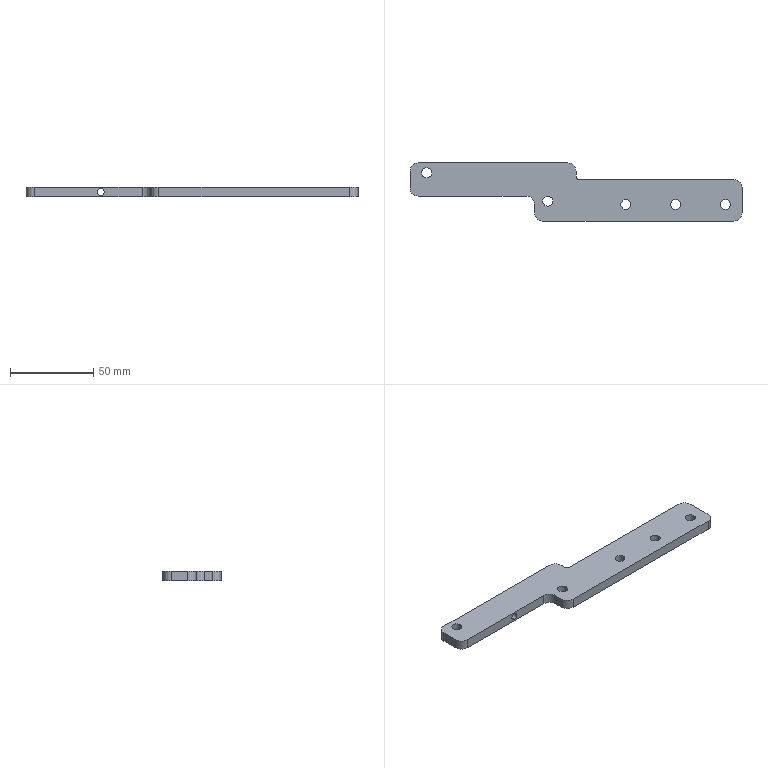Component | SolidWorks | Assembly5.1-1_MainTailstock.1-1 | 1 solid | 30 faces | box 200 x 35 x 6 mm | volume 27969 mm3 | cylinder 20 | plane 10 | commonest cylinder face diameters 6 x10 10 x7 4.2 x2 4 x1
build123d program:
from build123d import *

# Parameters (mm, degrees)
SKETCH1_R                  = 3
BOSS_EXTRUDE1_DEPTH        = 6
F_4_2_4_2_DIAMETER_HOLE1_D = 4.2


with BuildPart() as part:
    # Sketch1 → Boss-Extrude1 (new body)
    with BuildSketch(Plane.XY):
        with BuildLine():
            Line((-70, 20), (20, 20))
            ThreePointArc((20, 20), (23.536, 18.536), (25, 15))
            Line((25, 15), (25, 12))
            ThreePointArc((25, 12), (25.586, 10.586), (27, 10))
            Line((27, 10), (120, 10))
            ThreePointArc((120, 10), (123.536, 8.536), (125, 5))
            Line((125, 5), (125, -10))
            ThreePointArc((125, -10), (123.536, -13.536), (120, -15))
            Line((120, -15), (5, -15))
            ThreePointArc((5, -15), (1.464, -13.536), (0, -10))
            Line((0, -10), (0, -5))
            ThreePointArc((0, -5), (-1.464, -1.464), (-5, 0))
            Line((-5, 0), (-70, 0))
            ThreePointArc((-70, 0), (-73.536, 1.464), (-75, 5))
            Line((-75, 5), (-75, 15))
            ThreePointArc((-75, 15), (-73.536, 18.536), (-70, 20))
        make_face()
        with Locations((-65, 14)):
            Circle(SKETCH1_R, mode=Mode.SUBTRACT)
        with Locations((115, -5)):
            Circle(SKETCH1_R, mode=Mode.SUBTRACT)
        with Locations((85, -5)):
            Circle(SKETCH1_R, mode=Mode.SUBTRACT)
        with Locations((55, -5)):
            Circle(SKETCH1_R, mode=Mode.SUBTRACT)
        with Locations((8, -3)):
            Circle(SKETCH1_R, mode=Mode.SUBTRACT)
    extrude(amount=BOSS_EXTRUDE1_DEPTH)

    # 4.2 _4.2_ Diameter Hole1 (through all)
    with Locations(Plane(origin=(0, 20, 0), x_dir=(-1, 0, 0), z_dir=(0, 1, 0))):
        with Locations((30, 3)):
            Hole(F_4_2_4_2_DIAMETER_HOLE1_D / 2)


solid = part.part

# Placed as in the assembly
solid = solid.moved(Location((135, 150, -67.5), (0, 0, 0)))
STEP:
#1=COLOUR_RGB('',0.7922,0.8196,0.9333);
#2=FILL_AREA_STYLE_COLOUR('',#1);
#3=FILL_AREA_STYLE('',(#2));
#4=SURFACE_STYLE_FILL_AREA(#3);
#5=SURFACE_SIDE_STYLE('',(#4));
#6=SURFACE_STYLE_USAGE(.BOTH.,#5);
#7=PRESENTATION_STYLE_ASSIGNMENT((#6));
#8=CARTESIAN_POINT('',(4.134,5.906,-2.622));
#9=VERTEX_POINT('',#8);
#10=CARTESIAN_POINT('',(4.134,5.906,-2.457));
#11=VERTEX_POINT('',#10);
#12=CARTESIAN_POINT('',(4.134,5.906,-2.539));
#13=DIRECTION('',(-0.,1.,0.));
#14=DIRECTION('',(-1.,0.,0.));
#15=AXIS2_PLACEMENT_3D('',#12,#13,#14);
#16=CIRCLE('',#15,0.08268);
#17=EDGE_CURVE('',#9,#11,#16,.T.);
#18=ORIENTED_EDGE('',*,*,#17,.F.);
#19=CARTESIAN_POINT('',(4.134,6.693,-2.622));
#20=VERTEX_POINT('',#19);
#21=CARTESIAN_POINT('',(4.134,6.693,-2.622));
#22=DIRECTION('',(0.,1.,0.));
#23=VECTOR('',#22,39.37);
#24=LINE('',#21,#23);
#25=EDGE_CURVE('',#9,#20,#24,.T.);
#26=ORIENTED_EDGE('',*,*,#25,.T.);
#27=CARTESIAN_POINT('',(4.134,6.693,-2.457));
#28=VERTEX_POINT('',#27);
#29=CARTESIAN_POINT('',(4.134,6.693,-2.539));
#30=DIRECTION('',(0.,1.,0.));
#31=DIRECTION('',(0.,0.,1.));
#32=AXIS2_PLACEMENT_3D('',#29,#30,#31);
#33=CIRCLE('',#32,0.08268);
#34=EDGE_CURVE('',#20,#28,#33,.T.);
#35=ORIENTED_EDGE('',*,*,#34,.T.);
#36=CARTESIAN_POINT('',(4.134,6.693,-2.457));
#37=DIRECTION('',(0.,1.,0.));
#38=VECTOR('',#37,39.37);
#39=LINE('',#36,#38);
#40=EDGE_CURVE('',#11,#28,#39,.T.);
#41=ORIENTED_EDGE('',*,*,#40,.F.);
#42=EDGE_LOOP('',(#18,#26,#35,#41));
#43=FACE_OUTER_BOUND('',#42,.T.);
#44=CARTESIAN_POINT('',(4.134,6.693,-2.539));
#45=DIRECTION('',(0.,1.,0.));
#46=DIRECTION('',(0.,0.,1.));
#47=AXIS2_PLACEMENT_3D('',#44,#45,#46);
#48=CYLINDRICAL_SURFACE('',#47,0.08268);
#49=ADVANCED_FACE('',(#43),#48,.F.);
#50=CARTESIAN_POINT('',(5.512,5.787,-2.421));
#51=VERTEX_POINT('',#50);
#52=CARTESIAN_POINT('',(5.748,5.787,-2.421));
#53=VERTEX_POINT('',#52);
#54=CARTESIAN_POINT('',(5.63,5.787,-2.421));
#55=DIRECTION('',(0.,0.,1.));
#56=DIRECTION('',(1.,0.,0.));
#57=AXIS2_PLACEMENT_3D('',#54,#55,#56);
#58=CIRCLE('',#57,0.1181);
#59=EDGE_CURVE('',#51,#53,#58,.T.);
#60=ORIENTED_EDGE('',*,*,#59,.T.);
#61=CARTESIAN_POINT('',(5.748,5.787,-2.657));
#62=VERTEX_POINT('',#61);
#63=CARTESIAN_POINT('',(5.748,5.787,-2.421));
#64=DIRECTION('',(0.,0.,-1.));
#65=VECTOR('',#64,39.37);
#66=LINE('',#63,#65);
#67=EDGE_CURVE('',#53,#62,#66,.T.);
#68=ORIENTED_EDGE('',*,*,#67,.T.);
#69=CARTESIAN_POINT('',(5.512,5.787,-2.657));
#70=VERTEX_POINT('',#69);
#71=CARTESIAN_POINT('',(5.63,5.787,-2.657));
#72=DIRECTION('',(0.,0.,1.));
#73=DIRECTION('',(1.,0.,0.));
#74=AXIS2_PLACEMENT_3D('',#71,#72,#73);
#75=CIRCLE('',#74,0.1181);
#76=EDGE_CURVE('',#70,#62,#75,.T.);
#77=ORIENTED_EDGE('',*,*,#76,.F.);
#78=CARTESIAN_POINT('',(5.512,5.787,-2.421));
#79=DIRECTION('',(0.,0.,-1.));
#80=VECTOR('',#79,39.37);
#81=LINE('',#78,#80);
#82=EDGE_CURVE('',#51,#70,#81,.T.);
#83=ORIENTED_EDGE('',*,*,#82,.F.);
#84=EDGE_LOOP('',(#60,#68,#77,#83));
#85=FACE_OUTER_BOUND('',#84,.T.);
#86=CARTESIAN_POINT('',(5.63,5.787,-2.421));
#87=DIRECTION('',(0.,0.,-1.));
#88=DIRECTION('',(-1.,0.,0.));
#89=AXIS2_PLACEMENT_3D('',#86,#87,#88);
#90=CYLINDRICAL_SURFACE('',#89,0.1181);
#91=ADVANCED_FACE('',(#85),#90,.F.);
#92=CARTESIAN_POINT('',(7.362,5.709,-2.421));
#93=VERTEX_POINT('',#92);
#94=CARTESIAN_POINT('',(7.598,5.709,-2.421));
#95=VERTEX_POINT('',#94);
#96=CARTESIAN_POINT('',(7.48,5.709,-2.421));
#97=DIRECTION('',(0.,0.,1.));
#98=DIRECTION('',(1.,0.,0.));
#99=AXIS2_PLACEMENT_3D('',#96,#97,#98);
#100=CIRCLE('',#99,0.1181);
#101=EDGE_CURVE('',#93,#95,#100,.T.);
#102=ORIENTED_EDGE('',*,*,#101,.T.);
#103=CARTESIAN_POINT('',(7.598,5.709,-2.657));
#104=VERTEX_POINT('',#103);
#105=CARTESIAN_POINT('',(7.598,5.709,-2.421));
#106=DIRECTION('',(0.,0.,-1.));
#107=VECTOR('',#106,39.37);
#108=LINE('',#105,#107);
#109=EDGE_CURVE('',#95,#104,#108,.T.);
#110=ORIENTED_EDGE('',*,*,#109,.T.);
#111=CARTESIAN_POINT('',(7.362,5.709,-2.657));
#112=VERTEX_POINT('',#111);
#113=CARTESIAN_POINT('',(7.48,5.709,-2.657));
#114=DIRECTION('',(0.,0.,1.));
#115=DIRECTION('',(1.,0.,0.));
#116=AXIS2_PLACEMENT_3D('',#113,#114,#115);
#117=CIRCLE('',#116,0.1181);
#118=EDGE_CURVE('',#112,#104,#117,.T.);
#119=ORIENTED_EDGE('',*,*,#118,.F.);
#120=CARTESIAN_POINT('',(7.362,5.709,-2.421));
#121=DIRECTION('',(0.,0.,-1.));
#122=VECTOR('',#121,39.37);
#123=LINE('',#120,#122);
#124=EDGE_CURVE('',#93,#112,#123,.T.);
#125=ORIENTED_EDGE('',*,*,#124,.F.);
#126=EDGE_LOOP('',(#102,#110,#119,#125));
#127=FACE_OUTER_BOUND('',#126,.T.);
#128=CARTESIAN_POINT('',(7.48,5.709,-2.421));
#129=DIRECTION('',(0.,0.,-1.));
#130=DIRECTION('',(-1.,0.,0.));
#131=AXIS2_PLACEMENT_3D('',#128,#129,#130);
#132=CYLINDRICAL_SURFACE('',#131,0.1181);
#133=ADVANCED_FACE('',(#127),#132,.F.);
#134=CARTESIAN_POINT('',(8.543,5.709,-2.421));
#135=VERTEX_POINT('',#134);
#136=CARTESIAN_POINT('',(8.78,5.709,-2.421));
#137=VERTEX_POINT('',#136);
#138=CARTESIAN_POINT('',(8.661,5.709,-2.421));
#139=DIRECTION('',(0.,0.,1.));
#140=DIRECTION('',(1.,0.,0.));
#141=AXIS2_PLACEMENT_3D('',#138,#139,#140);
#142=CIRCLE('',#141,0.1181);
#143=EDGE_CURVE('',#135,#137,#142,.T.);
#144=ORIENTED_EDGE('',*,*,#143,.T.);
#145=CARTESIAN_POINT('',(8.78,5.709,-2.657));
#146=VERTEX_POINT('',#145);
#147=CARTESIAN_POINT('',(8.78,5.709,-2.421));
#148=DIRECTION('',(0.,0.,-1.));
#149=VECTOR('',#148,39.37);
#150=LINE('',#147,#149);
#151=EDGE_CURVE('',#137,#146,#150,.T.);
#152=ORIENTED_EDGE('',*,*,#151,.T.);
#153=CARTESIAN_POINT('',(8.543,5.709,-2.657));
#154=VERTEX_POINT('',#153);
#155=CARTESIAN_POINT('',(8.661,5.709,-2.657));
#156=DIRECTION('',(0.,0.,1.));
#157=DIRECTION('',(1.,0.,0.));
#158=AXIS2_PLACEMENT_3D('',#155,#156,#157);
#159=CIRCLE('',#158,0.1181);
#160=EDGE_CURVE('',#154,#146,#159,.T.);
#161=ORIENTED_EDGE('',*,*,#160,.F.);
#162=CARTESIAN_POINT('',(8.543,5.709,-2.421));
#163=DIRECTION('',(0.,0.,-1.));
#164=VECTOR('',#163,39.37);
#165=LINE('',#162,#164);
#166=EDGE_CURVE('',#135,#154,#165,.T.);
#167=ORIENTED_EDGE('',*,*,#166,.F.);
#168=EDGE_LOOP('',(#144,#152,#161,#167));
#169=FACE_OUTER_BOUND('',#168,.T.);
#170=CARTESIAN_POINT('',(8.661,5.709,-2.421));
#171=DIRECTION('',(0.,0.,-1.));
#172=DIRECTION('',(-1.,0.,0.));
#173=AXIS2_PLACEMENT_3D('',#170,#171,#172);
#174=CYLINDRICAL_SURFACE('',#173,0.1181);
#175=ADVANCED_FACE('',(#169),#174,.F.);
#176=CARTESIAN_POINT('',(9.724,5.709,-2.421));
#177=VERTEX_POINT('',#176);
#178=CARTESIAN_POINT('',(9.961,5.709,-2.421));
#179=VERTEX_POINT('',#178);
#180=CARTESIAN_POINT('',(9.843,5.709,-2.421));
#181=DIRECTION('',(0.,0.,1.));
#182=DIRECTION('',(1.,0.,0.));
#183=AXIS2_PLACEMENT_3D('',#180,#181,#182);
#184=CIRCLE('',#183,0.1181);
#185=EDGE_CURVE('',#177,#179,#184,.T.);
#186=ORIENTED_EDGE('',*,*,#185,.T.);
#187=CARTESIAN_POINT('',(9.961,5.709,-2.657));
#188=VERTEX_POINT('',#187);
#189=CARTESIAN_POINT('',(9.961,5.709,-2.421));
#190=DIRECTION('',(0.,0.,-1.));
#191=VECTOR('',#190,39.37);
#192=LINE('',#189,#191);
#193=EDGE_CURVE('',#179,#188,#192,.T.);
#194=ORIENTED_EDGE('',*,*,#193,.T.);
#195=CARTESIAN_POINT('',(9.724,5.709,-2.657));
#196=VERTEX_POINT('',#195);
#197=CARTESIAN_POINT('',(9.843,5.709,-2.657));
#198=DIRECTION('',(0.,0.,1.));
#199=DIRECTION('',(1.,0.,0.));
#200=AXIS2_PLACEMENT_3D('',#197,#198,#199);
#201=CIRCLE('',#200,0.1181);
#202=EDGE_CURVE('',#196,#188,#201,.T.);
#203=ORIENTED_EDGE('',*,*,#202,.F.);
#204=CARTESIAN_POINT('',(9.724,5.709,-2.421));
#205=DIRECTION('',(0.,0.,-1.));
#206=VECTOR('',#205,39.37);
#207=LINE('',#204,#206);
#208=EDGE_CURVE('',#177,#196,#207,.T.);
#209=ORIENTED_EDGE('',*,*,#208,.F.);
#210=EDGE_LOOP('',(#186,#194,#203,#209));
#211=FACE_OUTER_BOUND('',#210,.T.);
#212=CARTESIAN_POINT('',(9.843,5.709,-2.421));
#213=DIRECTION('',(0.,0.,-1.));
#214=DIRECTION('',(-1.,0.,0.));
#215=AXIS2_PLACEMENT_3D('',#212,#213,#214);
#216=CYLINDRICAL_SURFACE('',#215,0.1181);
#217=ADVANCED_FACE('',(#211),#216,.F.);
#218=CARTESIAN_POINT('',(2.638,6.457,-2.421));
#219=VERTEX_POINT('',#218);
#220=CARTESIAN_POINT('',(2.874,6.457,-2.421));
#221=VERTEX_POINT('',#220);
#222=CARTESIAN_POINT('',(2.756,6.457,-2.421));
#223=DIRECTION('',(0.,0.,1.));
#224=DIRECTION('',(1.,0.,0.));
#225=AXIS2_PLACEMENT_3D('',#222,#223,#224);
#226=CIRCLE('',#225,0.1181);
#227=EDGE_CURVE('',#219,#221,#226,.T.);
#228=ORIENTED_EDGE('',*,*,#227,.T.);
#229=CARTESIAN_POINT('',(2.874,6.457,-2.657));
#230=VERTEX_POINT('',#229);
#231=CARTESIAN_POINT('',(2.874,6.457,-2.421));
#232=DIRECTION('',(0.,0.,-1.));
#233=VECTOR('',#232,39.37);
#234=LINE('',#231,#233);
#235=EDGE_CURVE('',#221,#230,#234,.T.);
#236=ORIENTED_EDGE('',*,*,#235,.T.);
#237=CARTESIAN_POINT('',(2.638,6.457,-2.657));
#238=VERTEX_POINT('',#237);
#239=CARTESIAN_POINT('',(2.756,6.457,-2.657));
#240=DIRECTION('',(0.,0.,1.));
#241=DIRECTION('',(1.,0.,0.));
#242=AXIS2_PLACEMENT_3D('',#239,#240,#241);
#243=CIRCLE('',#242,0.1181);
#244=EDGE_CURVE('',#238,#230,#243,.T.);
#245=ORIENTED_EDGE('',*,*,#244,.F.);
#246=CARTESIAN_POINT('',(2.638,6.457,-2.421));
#247=DIRECTION('',(0.,0.,-1.));
#248=VECTOR('',#247,39.37);
#249=LINE('',#246,#248);
#250=EDGE_CURVE('',#219,#238,#249,.T.);
#251=ORIENTED_EDGE('',*,*,#250,.F.);
#252=EDGE_LOOP('',(#228,#236,#245,#251));
#253=FACE_OUTER_BOUND('',#252,.T.);
#254=CARTESIAN_POINT('',(2.756,6.457,-2.421));
#255=DIRECTION('',(0.,0.,-1.));
#256=DIRECTION('',(-1.,0.,0.));
#257=AXIS2_PLACEMENT_3D('',#254,#255,#256);
#258=CYLINDRICAL_SURFACE('',#257,0.1181);
#259=ADVANCED_FACE('',(#253),#258,.F.);
#260=ORIENTED_EDGE('',*,*,#101,.F.);
#261=CARTESIAN_POINT('',(7.48,5.709,-2.421));
#262=DIRECTION('',(0.,0.,1.));
#263=DIRECTION('',(1.,0.,0.));
#264=AXIS2_PLACEMENT_3D('',#261,#262,#263);
#265=CIRCLE('',#264,0.1181);
#266=EDGE_CURVE('',#95,#93,#265,.T.);
#267=ORIENTED_EDGE('',*,*,#266,.F.);
#268=EDGE_LOOP('',(#260,#267));
#269=FACE_BOUND('',#268,.T.);
#270=ORIENTED_EDGE('',*,*,#185,.F.);
#271=CARTESIAN_POINT('',(9.843,5.709,-2.421));
#272=DIRECTION('',(0.,0.,1.));
#273=DIRECTION('',(1.,0.,0.));
#274=AXIS2_PLACEMENT_3D('',#271,#272,#273);
#275=CIRCLE('',#274,0.1181);
#276=EDGE_CURVE('',#179,#177,#275,.T.);
#277=ORIENTED_EDGE('',*,*,#276,.F.);
#278=EDGE_LOOP('',(#270,#277));
#279=FACE_BOUND('',#278,.T.);
#280=CARTESIAN_POINT('',(10.039,5.315,-2.421));
#281=VERTEX_POINT('',#280);
#282=CARTESIAN_POINT('',(10.236,5.512,-2.421));
#283=VERTEX_POINT('',#282);
#284=CARTESIAN_POINT('',(10.039,5.512,-2.421));
#285=DIRECTION('',(0.,0.,1.));
#286=DIRECTION('',(1.,0.,0.));
#287=AXIS2_PLACEMENT_3D('',#284,#285,#286);
#288=CIRCLE('',#287,0.1969);
#289=EDGE_CURVE('',#281,#283,#288,.T.);
#290=ORIENTED_EDGE('',*,*,#289,.T.);
#291=CARTESIAN_POINT('',(10.236,6.102,-2.421));
#292=VERTEX_POINT('',#291);
#293=CARTESIAN_POINT('',(10.236,6.102,-2.421));
#294=DIRECTION('',(0.,1.,0.));
#295=VECTOR('',#294,39.37);
#296=LINE('',#293,#295);
#297=EDGE_CURVE('',#283,#292,#296,.T.);
#298=ORIENTED_EDGE('',*,*,#297,.T.);
#299=CARTESIAN_POINT('',(10.039,6.299,-2.421));
#300=VERTEX_POINT('',#299);
#301=CARTESIAN_POINT('',(10.039,6.102,-2.421));
#302=DIRECTION('',(0.,0.,1.));
#303=DIRECTION('',(1.,0.,0.));
#304=AXIS2_PLACEMENT_3D('',#301,#302,#303);
#305=CIRCLE('',#304,0.1969);
#306=EDGE_CURVE('',#292,#300,#305,.T.);
#307=ORIENTED_EDGE('',*,*,#306,.T.);
#308=CARTESIAN_POINT('',(6.378,6.299,-2.421));
#309=VERTEX_POINT('',#308);
#310=CARTESIAN_POINT('',(6.378,6.299,-2.421));
#311=DIRECTION('',(-1.,-0.,0.));
#312=VECTOR('',#311,39.37);
#313=LINE('',#310,#312);
#314=EDGE_CURVE('',#300,#309,#313,.T.);
#315=ORIENTED_EDGE('',*,*,#314,.T.);
#316=CARTESIAN_POINT('',(6.299,6.378,-2.421));
#317=VERTEX_POINT('',#316);
#318=CARTESIAN_POINT('',(6.378,6.378,-2.421));
#319=DIRECTION('',(0.,0.,-1.));
#320=DIRECTION('',(-1.,0.,0.));
#321=AXIS2_PLACEMENT_3D('',#318,#319,#320);
#322=CIRCLE('',#321,0.07874);
#323=EDGE_CURVE('',#309,#317,#322,.T.);
#324=ORIENTED_EDGE('',*,*,#323,.T.);
#325=CARTESIAN_POINT('',(6.299,6.496,-2.421));
#326=VERTEX_POINT('',#325);
#327=CARTESIAN_POINT('',(6.299,6.496,-2.421));
#328=DIRECTION('',(0.,1.,0.));
#329=VECTOR('',#328,39.37);
#330=LINE('',#327,#329);
#331=EDGE_CURVE('',#317,#326,#330,.T.);
#332=ORIENTED_EDGE('',*,*,#331,.T.);
#333=CARTESIAN_POINT('',(6.102,6.693,-2.421));
#334=VERTEX_POINT('',#333);
#335=CARTESIAN_POINT('',(6.102,6.496,-2.421));
#336=DIRECTION('',(0.,0.,1.));
#337=DIRECTION('',(1.,0.,0.));
#338=AXIS2_PLACEMENT_3D('',#335,#336,#337);
#339=CIRCLE('',#338,0.1969);
#340=EDGE_CURVE('',#326,#334,#339,.T.);
#341=ORIENTED_EDGE('',*,*,#340,.T.);
#342=CARTESIAN_POINT('',(2.559,6.693,-2.421));
#343=VERTEX_POINT('',#342);
#344=CARTESIAN_POINT('',(2.559,6.693,-2.421));
#345=DIRECTION('',(-1.,0.,0.));
#346=VECTOR('',#345,39.37);
#347=LINE('',#344,#346);
#348=EDGE_CURVE('',#334,#343,#347,.T.);
#349=ORIENTED_EDGE('',*,*,#348,.T.);
#350=CARTESIAN_POINT('',(2.362,6.496,-2.421));
#351=VERTEX_POINT('',#350);
#352=CARTESIAN_POINT('',(2.559,6.496,-2.421));
#353=DIRECTION('',(0.,0.,1.));
#354=DIRECTION('',(1.,0.,0.));
#355=AXIS2_PLACEMENT_3D('',#352,#353,#354);
#356=CIRCLE('',#355,0.1969);
#357=EDGE_CURVE('',#343,#351,#356,.T.);
#358=ORIENTED_EDGE('',*,*,#357,.T.);
#359=CARTESIAN_POINT('',(2.362,6.102,-2.421));
#360=VERTEX_POINT('',#359);
#361=CARTESIAN_POINT('',(2.362,6.102,-2.421));
#362=DIRECTION('',(0.,-1.,0.));
#363=VECTOR('',#362,39.37);
#364=LINE('',#361,#363);
#365=EDGE_CURVE('',#351,#360,#364,.T.);
#366=ORIENTED_EDGE('',*,*,#365,.T.);
#367=CARTESIAN_POINT('',(2.559,5.906,-2.421));
#368=VERTEX_POINT('',#367);
#369=CARTESIAN_POINT('',(2.559,6.102,-2.421));
#370=DIRECTION('',(0.,0.,1.));
#371=DIRECTION('',(-1.,0.,0.));
#372=AXIS2_PLACEMENT_3D('',#369,#370,#371);
#373=CIRCLE('',#372,0.1969);
#374=EDGE_CURVE('',#360,#368,#373,.T.);
#375=ORIENTED_EDGE('',*,*,#374,.T.);
#376=CARTESIAN_POINT('',(5.118,5.906,-2.421));
#377=VERTEX_POINT('',#376);
#378=CARTESIAN_POINT('',(5.118,5.906,-2.421));
#379=DIRECTION('',(1.,0.,0.));
#380=VECTOR('',#379,39.37);
#381=LINE('',#378,#380);
#382=EDGE_CURVE('',#368,#377,#381,.T.);
#383=ORIENTED_EDGE('',*,*,#382,.T.);
#384=CARTESIAN_POINT('',(5.315,5.709,-2.421));
#385=VERTEX_POINT('',#384);
#386=CARTESIAN_POINT('',(5.118,5.709,-2.421));
#387=DIRECTION('',(0.,0.,-1.));
#388=DIRECTION('',(1.,0.,0.));
#389=AXIS2_PLACEMENT_3D('',#386,#387,#388);
#390=CIRCLE('',#389,0.1969);
#391=EDGE_CURVE('',#377,#385,#390,.T.);
#392=ORIENTED_EDGE('',*,*,#391,.T.);
#393=CARTESIAN_POINT('',(5.315,5.512,-2.421));
#394=VERTEX_POINT('',#393);
#395=CARTESIAN_POINT('',(5.315,5.512,-2.421));
#396=DIRECTION('',(0.,-1.,0.));
#397=VECTOR('',#396,39.37);
#398=LINE('',#395,#397);
#399=EDGE_CURVE('',#385,#394,#398,.T.);
#400=ORIENTED_EDGE('',*,*,#399,.T.);
#401=CARTESIAN_POINT('',(5.512,5.315,-2.421));
#402=VERTEX_POINT('',#401);
#403=CARTESIAN_POINT('',(5.512,5.512,-2.421));
#404=DIRECTION('',(0.,0.,1.));
#405=DIRECTION('',(-1.,0.,0.));
#406=AXIS2_PLACEMENT_3D('',#403,#404,#405);
#407=CIRCLE('',#406,0.1969);
#408=EDGE_CURVE('',#394,#402,#407,.T.);
#409=ORIENTED_EDGE('',*,*,#408,.T.);
#410=CARTESIAN_POINT('',(10.039,5.315,-2.421));
#411=DIRECTION('',(1.,0.,0.));
#412=VECTOR('',#411,39.37);
#413=LINE('',#410,#412);
#414=EDGE_CURVE('',#402,#281,#413,.T.);
#415=ORIENTED_EDGE('',*,*,#414,.T.);
#416=EDGE_LOOP('',(#290,#298,#307,#315,#324,#332,#341,#349,#358,#366,#375,#383,#392,#400,#409,#415));
#417=FACE_OUTER_BOUND('',#416,.T.);
#418=ORIENTED_EDGE('',*,*,#227,.F.);
#419=CARTESIAN_POINT('',(2.756,6.457,-2.421));
#420=DIRECTION('',(0.,0.,1.));
#421=DIRECTION('',(1.,0.,0.));
#422=AXIS2_PLACEMENT_3D('',#419,#420,#421);
#423=CIRCLE('',#422,0.1181);
#424=EDGE_CURVE('',#221,#219,#423,.T.);
#425=ORIENTED_EDGE('',*,*,#424,.F.);
#426=EDGE_LOOP('',(#418,#425));
#427=FACE_BOUND('',#426,.T.);
#428=ORIENTED_EDGE('',*,*,#143,.F.);
#429=CARTESIAN_POINT('',(8.661,5.709,-2.421));
#430=DIRECTION('',(0.,0.,1.));
#431=DIRECTION('',(1.,0.,0.));
#432=AXIS2_PLACEMENT_3D('',#429,#430,#431);
#433=CIRCLE('',#432,0.1181);
#434=EDGE_CURVE('',#137,#135,#433,.T.);
#435=ORIENTED_EDGE('',*,*,#434,.F.);
#436=EDGE_LOOP('',(#428,#435));
#437=FACE_BOUND('',#436,.T.);
#438=ORIENTED_EDGE('',*,*,#59,.F.);
#439=CARTESIAN_POINT('',(5.63,5.787,-2.421));
#440=DIRECTION('',(0.,0.,1.));
#441=DIRECTION('',(1.,0.,0.));
#442=AXIS2_PLACEMENT_3D('',#439,#440,#441);
#443=CIRCLE('',#442,0.1181);
#444=EDGE_CURVE('',#53,#51,#443,.T.);
#445=ORIENTED_EDGE('',*,*,#444,.F.);
#446=EDGE_LOOP('',(#438,#445));
#447=FACE_BOUND('',#446,.T.);
#448=CARTESIAN_POINT('',(10.039,5.512,-2.421));
#449=DIRECTION('',(0.,0.,1.));
#450=DIRECTION('',(1.,0.,0.));
#451=AXIS2_PLACEMENT_3D('',#448,#449,#450);
#452=PLANE('',#451);
#453=ADVANCED_FACE('',(#269,#279,#417,#427,#437,#447),#452,.T.);
#454=ORIENTED_EDGE('',*,*,#118,.T.);
#455=CARTESIAN_POINT('',(7.48,5.709,-2.657));
#456=DIRECTION('',(0.,0.,1.));
#457=DIRECTION('',(1.,0.,0.));
#458=AXIS2_PLACEMENT_3D('',#455,#456,#457);
#459=CIRCLE('',#458,0.1181);
#460=EDGE_CURVE('',#104,#112,#459,.T.);
#461=ORIENTED_EDGE('',*,*,#460,.T.);
#462=EDGE_LOOP('',(#454,#461));
#463=FACE_BOUND('',#462,.T.);
#464=ORIENTED_EDGE('',*,*,#202,.T.);
#465=CARTESIAN_POINT('',(9.843,5.709,-2.657));
#466=DIRECTION('',(0.,0.,1.));
#467=DIRECTION('',(1.,0.,0.));
#468=AXIS2_PLACEMENT_3D('',#465,#466,#467);
#469=CIRCLE('',#468,0.1181);
#470=EDGE_CURVE('',#188,#196,#469,.T.);
#471=ORIENTED_EDGE('',*,*,#470,.T.);
#472=EDGE_LOOP('',(#464,#471));
#473=FACE_BOUND('',#472,.T.);
#474=CARTESIAN_POINT('',(10.039,5.315,-2.657));
#475=VERTEX_POINT('',#474);
#476=CARTESIAN_POINT('',(10.236,5.512,-2.657));
#477=VERTEX_POINT('',#476);
#478=CARTESIAN_POINT('',(10.039,5.512,-2.657));
#479=DIRECTION('',(0.,0.,1.));
#480=DIRECTION('',(1.,0.,0.));
#481=AXIS2_PLACEMENT_3D('',#478,#479,#480);
#482=CIRCLE('',#481,0.1969);
#483=EDGE_CURVE('',#475,#477,#482,.T.);
#484=ORIENTED_EDGE('',*,*,#483,.F.);
#485=CARTESIAN_POINT('',(5.512,5.315,-2.657));
#486=VERTEX_POINT('',#485);
#487=CARTESIAN_POINT('',(10.039,5.315,-2.657));
#488=DIRECTION('',(1.,0.,0.));
#489=VECTOR('',#488,39.37);
#490=LINE('',#487,#489);
#491=EDGE_CURVE('',#486,#475,#490,.T.);
#492=ORIENTED_EDGE('',*,*,#491,.F.);
#493=CARTESIAN_POINT('',(5.315,5.512,-2.657));
#494=VERTEX_POINT('',#493);
#495=CARTESIAN_POINT('',(5.512,5.512,-2.657));
#496=DIRECTION('',(0.,0.,1.));
#497=DIRECTION('',(-1.,0.,0.));
#498=AXIS2_PLACEMENT_3D('',#495,#496,#497);
#499=CIRCLE('',#498,0.1969);
#500=EDGE_CURVE('',#494,#486,#499,.T.);
#501=ORIENTED_EDGE('',*,*,#500,.F.);
#502=CARTESIAN_POINT('',(5.315,5.709,-2.657));
#503=VERTEX_POINT('',#502);
#504=CARTESIAN_POINT('',(5.315,5.512,-2.657));
#505=DIRECTION('',(0.,-1.,0.));
#506=VECTOR('',#505,39.37);
#507=LINE('',#504,#506);
#508=EDGE_CURVE('',#503,#494,#507,.T.);
#509=ORIENTED_EDGE('',*,*,#508,.F.);
#510=CARTESIAN_POINT('',(5.118,5.906,-2.657));
#511=VERTEX_POINT('',#510);
#512=CARTESIAN_POINT('',(5.118,5.709,-2.657));
#513=DIRECTION('',(0.,0.,-1.));
#514=DIRECTION('',(1.,0.,0.));
#515=AXIS2_PLACEMENT_3D('',#512,#513,#514);
#516=CIRCLE('',#515,0.1969);
#517=EDGE_CURVE('',#511,#503,#516,.T.);
#518=ORIENTED_EDGE('',*,*,#517,.F.);
#519=CARTESIAN_POINT('',(2.559,5.906,-2.657));
#520=VERTEX_POINT('',#519);
#521=CARTESIAN_POINT('',(5.118,5.906,-2.657));
#522=DIRECTION('',(1.,0.,0.));
#523=VECTOR('',#522,39.37);
#524=LINE('',#521,#523);
#525=EDGE_CURVE('',#520,#511,#524,.T.);
#526=ORIENTED_EDGE('',*,*,#525,.F.);
#527=CARTESIAN_POINT('',(2.362,6.102,-2.657));
#528=VERTEX_POINT('',#527);
#529=CARTESIAN_POINT('',(2.559,6.102,-2.657));
#530=DIRECTION('',(0.,0.,1.));
#531=DIRECTION('',(-1.,0.,0.));
#532=AXIS2_PLACEMENT_3D('',#529,#530,#531);
#533=CIRCLE('',#532,0.1969);
#534=EDGE_CURVE('',#528,#520,#533,.T.);
#535=ORIENTED_EDGE('',*,*,#534,.F.);
#536=CARTESIAN_POINT('',(2.362,6.496,-2.657));
#537=VERTEX_POINT('',#536);
#538=CARTESIAN_POINT('',(2.362,6.102,-2.657));
#539=DIRECTION('',(0.,-1.,0.));
#540=VECTOR('',#539,39.37);
#541=LINE('',#538,#540);
#542=EDGE_CURVE('',#537,#528,#541,.T.);
#543=ORIENTED_EDGE('',*,*,#542,.F.);
#544=CARTESIAN_POINT('',(2.559,6.693,-2.657));
#545=VERTEX_POINT('',#544);
#546=CARTESIAN_POINT('',(2.559,6.496,-2.657));
#547=DIRECTION('',(0.,0.,1.));
#548=DIRECTION('',(1.,0.,0.));
#549=AXIS2_PLACEMENT_3D('',#546,#547,#548);
#550=CIRCLE('',#549,0.1969);
#551=EDGE_CURVE('',#545,#537,#550,.T.);
#552=ORIENTED_EDGE('',*,*,#551,.F.);
#553=CARTESIAN_POINT('',(6.102,6.693,-2.657));
#554=VERTEX_POINT('',#553);
#555=CARTESIAN_POINT('',(2.559,6.693,-2.657));
#556=DIRECTION('',(-1.,0.,0.));
#557=VECTOR('',#556,39.37);
#558=LINE('',#555,#557);
#559=EDGE_CURVE('',#554,#545,#558,.T.);
#560=ORIENTED_EDGE('',*,*,#559,.F.);
#561=CARTESIAN_POINT('',(6.299,6.496,-2.657));
#562=VERTEX_POINT('',#561);
#563=CARTESIAN_POINT('',(6.102,6.496,-2.657));
#564=DIRECTION('',(0.,0.,1.));
#565=DIRECTION('',(1.,0.,0.));
#566=AXIS2_PLACEMENT_3D('',#563,#564,#565);
#567=CIRCLE('',#566,0.1969);
#568=EDGE_CURVE('',#562,#554,#567,.T.);
#569=ORIENTED_EDGE('',*,*,#568,.F.);
#570=CARTESIAN_POINT('',(6.299,6.378,-2.657));
#571=VERTEX_POINT('',#570);
#572=CARTESIAN_POINT('',(6.299,6.496,-2.657));
#573=DIRECTION('',(0.,1.,0.));
#574=VECTOR('',#573,39.37);
#575=LINE('',#572,#574);
#576=EDGE_CURVE('',#571,#562,#575,.T.);
#577=ORIENTED_EDGE('',*,*,#576,.F.);
#578=CARTESIAN_POINT('',(6.378,6.299,-2.657));
#579=VERTEX_POINT('',#578);
#580=CARTESIAN_POINT('',(6.378,6.378,-2.657));
#581=DIRECTION('',(0.,0.,-1.));
#582=DIRECTION('',(-1.,0.,0.));
#583=AXIS2_PLACEMENT_3D('',#580,#581,#582);
#584=CIRCLE('',#583,0.07874);
#585=EDGE_CURVE('',#579,#571,#584,.T.);
#586=ORIENTED_EDGE('',*,*,#585,.F.);
#587=CARTESIAN_POINT('',(10.039,6.299,-2.657));
#588=VERTEX_POINT('',#587);
#589=CARTESIAN_POINT('',(6.378,6.299,-2.657));
#590=DIRECTION('',(-1.,-0.,0.));
#591=VECTOR('',#590,39.37);
#592=LINE('',#589,#591);
#593=EDGE_CURVE('',#588,#579,#592,.T.);
#594=ORIENTED_EDGE('',*,*,#593,.F.);
#595=CARTESIAN_POINT('',(10.236,6.102,-2.657));
#596=VERTEX_POINT('',#595);
#597=CARTESIAN_POINT('',(10.039,6.102,-2.657));
#598=DIRECTION('',(0.,0.,1.));
#599=DIRECTION('',(1.,0.,0.));
#600=AXIS2_PLACEMENT_3D('',#597,#598,#599);
#601=CIRCLE('',#600,0.1969);
#602=EDGE_CURVE('',#596,#588,#601,.T.);
#603=ORIENTED_EDGE('',*,*,#602,.F.);
#604=CARTESIAN_POINT('',(10.236,6.102,-2.657));
#605=DIRECTION('',(0.,1.,0.));
#606=VECTOR('',#605,39.37);
#607=LINE('',#604,#606);
#608=EDGE_CURVE('',#477,#596,#607,.T.);
#609=ORIENTED_EDGE('',*,*,#608,.F.);
#610=EDGE_LOOP('',(#484,#492,#501,#509,#518,#526,#535,#543,#552,#560,#569,#577,#586,#594,#603,#609));
#611=FACE_OUTER_BOUND('',#610,.T.);
#612=ORIENTED_EDGE('',*,*,#244,.T.);
#613=CARTESIAN_POINT('',(2.756,6.457,-2.657));
#614=DIRECTION('',(0.,0.,1.));
#615=DIRECTION('',(1.,0.,0.));
#616=AXIS2_PLACEMENT_3D('',#613,#614,#615);
#617=CIRCLE('',#616,0.1181);
#618=EDGE_CURVE('',#230,#238,#617,.T.);
#619=ORIENTED_EDGE('',*,*,#618,.T.);
#620=EDGE_LOOP('',(#612,#619));
#621=FACE_BOUND('',#620,.T.);
#622=ORIENTED_EDGE('',*,*,#160,.T.);
#623=CARTESIAN_POINT('',(8.661,5.709,-2.657));
#624=DIRECTION('',(0.,0.,1.));
#625=DIRECTION('',(1.,0.,0.));
#626=AXIS2_PLACEMENT_3D('',#623,#624,#625);
#627=CIRCLE('',#626,0.1181);
#628=EDGE_CURVE('',#146,#154,#627,.T.);
#629=ORIENTED_EDGE('',*,*,#628,.T.);
#630=EDGE_LOOP('',(#622,#629));
#631=FACE_BOUND('',#630,.T.);
#632=ORIENTED_EDGE('',*,*,#76,.T.);
#633=CARTESIAN_POINT('',(5.63,5.787,-2.657));
#634=DIRECTION('',(0.,0.,1.));
#635=DIRECTION('',(1.,0.,0.));
#636=AXIS2_PLACEMENT_3D('',#633,#634,#635);
#637=CIRCLE('',#636,0.1181);
#638=EDGE_CURVE('',#62,#70,#637,.T.);
#639=ORIENTED_EDGE('',*,*,#638,.T.);
#640=EDGE_LOOP('',(#632,#639));
#641=FACE_BOUND('',#640,.T.);
#642=CARTESIAN_POINT('',(10.039,5.512,-2.657));
#643=DIRECTION('',(0.,0.,1.));
#644=DIRECTION('',(1.,0.,0.));
#645=AXIS2_PLACEMENT_3D('',#642,#643,#644);
#646=PLANE('',#645);
#647=ADVANCED_FACE('',(#463,#473,#611,#621,#631,#641),#646,.F.);
#648=ORIENTED_EDGE('',*,*,#483,.T.);
#649=CARTESIAN_POINT('',(10.236,5.512,-2.421));
#650=DIRECTION('',(0.,0.,-1.));
#651=VECTOR('',#650,39.37);
#652=LINE('',#649,#651);
#653=EDGE_CURVE('',#283,#477,#652,.T.);
#654=ORIENTED_EDGE('',*,*,#653,.F.);
#655=ORIENTED_EDGE('',*,*,#289,.F.);
#656=CARTESIAN_POINT('',(10.039,5.315,-2.421));
#657=DIRECTION('',(0.,0.,-1.));
#658=VECTOR('',#657,39.37);
#659=LINE('',#656,#658);
#660=EDGE_CURVE('',#281,#475,#659,.T.);
#661=ORIENTED_EDGE('',*,*,#660,.T.);
#662=EDGE_LOOP('',(#648,#654,#655,#661));
#663=FACE_OUTER_BOUND('',#662,.T.);
#664=CARTESIAN_POINT('',(10.039,5.512,-2.421));
#665=DIRECTION('',(0.,0.,-1.));
#666=DIRECTION('',(-1.,0.,0.));
#667=AXIS2_PLACEMENT_3D('',#664,#665,#666);
#668=CYLINDRICAL_SURFACE('',#667,0.1969);
#669=ADVANCED_FACE('',(#663),#668,.T.);
#670=ORIENTED_EDGE('',*,*,#608,.T.);
#671=CARTESIAN_POINT('',(10.236,6.102,-2.421));
#672=DIRECTION('',(0.,0.,-1.));
#673=VECTOR('',#672,39.37);
#674=LINE('',#671,#673);
#675=EDGE_CURVE('',#292,#596,#674,.T.);
#676=ORIENTED_EDGE('',*,*,#675,.F.);
#677=ORIENTED_EDGE('',*,*,#297,.F.);
#678=ORIENTED_EDGE('',*,*,#653,.T.);
#679=EDGE_LOOP('',(#670,#676,#677,#678));
#680=FACE_OUTER_BOUND('',#679,.T.);
#681=CARTESIAN_POINT('',(10.236,6.102,-2.421));
#682=DIRECTION('',(-1.,0.,0.));
#683=DIRECTION('',(0.,0.,1.));
#684=AXIS2_PLACEMENT_3D('',#681,#682,#683);
#685=PLANE('',#684);
#686=ADVANCED_FACE('',(#680),#685,.F.);
#687=ORIENTED_EDGE('',*,*,#602,.T.);
#688=CARTESIAN_POINT('',(10.039,6.299,-2.421));
#689=DIRECTION('',(0.,0.,-1.));
#690=VECTOR('',#689,39.37);
#691=LINE('',#688,#690);
#692=EDGE_CURVE('',#300,#588,#691,.T.);
#693=ORIENTED_EDGE('',*,*,#692,.F.);
#694=ORIENTED_EDGE('',*,*,#306,.F.);
#695=ORIENTED_EDGE('',*,*,#675,.T.);
#696=EDGE_LOOP('',(#687,#693,#694,#695));
#697=FACE_OUTER_BOUND('',#696,.T.);
#698=CARTESIAN_POINT('',(10.039,6.102,-2.421));
#699=DIRECTION('',(0.,0.,-1.));
#700=DIRECTION('',(-1.,0.,0.));
#701=AXIS2_PLACEMENT_3D('',#698,#699,#700);
#702=CYLINDRICAL_SURFACE('',#701,0.1969);
#703=ADVANCED_FACE('',(#697),#702,.T.);
#704=ORIENTED_EDGE('',*,*,#593,.T.);
#705=CARTESIAN_POINT('',(6.378,6.299,-2.421));
#706=DIRECTION('',(0.,0.,-1.));
#707=VECTOR('',#706,39.37);
#708=LINE('',#705,#707);
#709=EDGE_CURVE('',#309,#579,#708,.T.);
#710=ORIENTED_EDGE('',*,*,#709,.F.);
#711=ORIENTED_EDGE('',*,*,#314,.F.);
#712=ORIENTED_EDGE('',*,*,#692,.T.);
#713=EDGE_LOOP('',(#704,#710,#711,#712));
#714=FACE_OUTER_BOUND('',#713,.T.);
#715=CARTESIAN_POINT('',(6.378,6.299,-2.421));
#716=DIRECTION('',(0.,-1.,0.));
#717=DIRECTION('',(1.,0.,0.));
#718=AXIS2_PLACEMENT_3D('',#715,#716,#717);
#719=PLANE('',#718);
#720=ADVANCED_FACE('',(#714),#719,.F.);
#721=ORIENTED_EDGE('',*,*,#585,.T.);
#722=CARTESIAN_POINT('',(6.299,6.378,-2.421));
#723=DIRECTION('',(0.,0.,-1.));
#724=VECTOR('',#723,39.37);
#725=LINE('',#722,#724);
#726=EDGE_CURVE('',#317,#571,#725,.T.);
#727=ORIENTED_EDGE('',*,*,#726,.F.);
#728=ORIENTED_EDGE('',*,*,#323,.F.);
#729=ORIENTED_EDGE('',*,*,#709,.T.);
#730=EDGE_LOOP('',(#721,#727,#728,#729));
#731=FACE_OUTER_BOUND('',#730,.T.);
#732=CARTESIAN_POINT('',(6.378,6.378,-2.421));
#733=DIRECTION('',(0.,0.,-1.));
#734=DIRECTION('',(-1.,0.,0.));
#735=AXIS2_PLACEMENT_3D('',#732,#733,#734);
#736=CYLINDRICAL_SURFACE('',#735,0.07874);
#737=ADVANCED_FACE('',(#731),#736,.F.);
#738=ORIENTED_EDGE('',*,*,#576,.T.);
#739=CARTESIAN_POINT('',(6.299,6.496,-2.421));
#740=DIRECTION('',(0.,0.,-1.));
#741=VECTOR('',#740,39.37);
#742=LINE('',#739,#741);
#743=EDGE_CURVE('',#326,#562,#742,.T.);
#744=ORIENTED_EDGE('',*,*,#743,.F.);
#745=ORIENTED_EDGE('',*,*,#331,.F.);
#746=ORIENTED_EDGE('',*,*,#726,.T.);
#747=EDGE_LOOP('',(#738,#744,#745,#746));
#748=FACE_OUTER_BOUND('',#747,.T.);
#749=CARTESIAN_POINT('',(6.299,6.496,-2.421));
#750=DIRECTION('',(-1.,0.,0.));
#751=DIRECTION('',(0.,0.,1.));
#752=AXIS2_PLACEMENT_3D('',#749,#750,#751);
#753=PLANE('',#752);
#754=ADVANCED_FACE('',(#748),#753,.F.);
#755=ORIENTED_EDGE('',*,*,#568,.T.);
#756=CARTESIAN_POINT('',(6.102,6.693,-2.421));
#757=DIRECTION('',(0.,0.,-1.));
#758=VECTOR('',#757,39.37);
#759=LINE('',#756,#758);
#760=EDGE_CURVE('',#334,#554,#759,.T.);
#761=ORIENTED_EDGE('',*,*,#760,.F.);
#762=ORIENTED_EDGE('',*,*,#340,.F.);
#763=ORIENTED_EDGE('',*,*,#743,.T.);
#764=EDGE_LOOP('',(#755,#761,#762,#763));
#765=FACE_OUTER_BOUND('',#764,.T.);
#766=CARTESIAN_POINT('',(6.102,6.496,-2.421));
#767=DIRECTION('',(0.,0.,-1.));
#768=DIRECTION('',(-1.,0.,0.));
#769=AXIS2_PLACEMENT_3D('',#766,#767,#768);
#770=CYLINDRICAL_SURFACE('',#769,0.1969);
#771=ADVANCED_FACE('',(#765),#770,.T.);
#772=CARTESIAN_POINT('',(4.134,6.693,-2.539));
#773=DIRECTION('',(0.,1.,0.));
#774=DIRECTION('',(0.,0.,1.));
#775=AXIS2_PLACEMENT_3D('',#772,#773,#774);
#776=CIRCLE('',#775,0.08268);
#777=EDGE_CURVE('',#28,#20,#776,.T.);
#778=ORIENTED_EDGE('',*,*,#777,.F.);
#779=ORIENTED_EDGE('',*,*,#34,.F.);
#780=EDGE_LOOP('',(#778,#779));
#781=FACE_BOUND('',#780,.T.);
#782=ORIENTED_EDGE('',*,*,#559,.T.);
#783=CARTESIAN_POINT('',(2.559,6.693,-2.421));
#784=DIRECTION('',(0.,0.,-1.));
#785=VECTOR('',#784,39.37);
#786=LINE('',#783,#785);
#787=EDGE_CURVE('',#343,#545,#786,.T.);
#788=ORIENTED_EDGE('',*,*,#787,.F.);
#789=ORIENTED_EDGE('',*,*,#348,.F.);
#790=ORIENTED_EDGE('',*,*,#760,.T.);
#791=EDGE_LOOP('',(#782,#788,#789,#790));
#792=FACE_OUTER_BOUND('',#791,.T.);
#793=CARTESIAN_POINT('',(2.559,6.693,-2.421));
#794=DIRECTION('',(-0.,-1.,0.));
#795=DIRECTION('',(1.,-0.,0.));
#796=AXIS2_PLACEMENT_3D('',#793,#794,#795);
#797=PLANE('',#796);
#798=ADVANCED_FACE('',(#781,#792),#797,.F.);
#799=ORIENTED_EDGE('',*,*,#551,.T.);
#800=CARTESIAN_POINT('',(2.362,6.496,-2.421));
#801=DIRECTION('',(0.,0.,-1.));
#802=VECTOR('',#801,39.37);
#803=LINE('',#800,#802);
#804=EDGE_CURVE('',#351,#537,#803,.T.);
#805=ORIENTED_EDGE('',*,*,#804,.F.);
#806=ORIENTED_EDGE('',*,*,#357,.F.);
#807=ORIENTED_EDGE('',*,*,#787,.T.);
#808=EDGE_LOOP('',(#799,#805,#806,#807));
#809=FACE_OUTER_BOUND('',#808,.T.);
#810=CARTESIAN_POINT('',(2.559,6.496,-2.421));
#811=DIRECTION('',(0.,0.,-1.));
#812=DIRECTION('',(-1.,0.,0.));
#813=AXIS2_PLACEMENT_3D('',#810,#811,#812);
#814=CYLINDRICAL_SURFACE('',#813,0.1969);
#815=ADVANCED_FACE('',(#809),#814,.T.);
#816=ORIENTED_EDGE('',*,*,#542,.T.);
#817=CARTESIAN_POINT('',(2.362,6.102,-2.421));
#818=DIRECTION('',(0.,0.,-1.));
#819=VECTOR('',#818,39.37);
#820=LINE('',#817,#819);
#821=EDGE_CURVE('',#360,#528,#820,.T.);
#822=ORIENTED_EDGE('',*,*,#821,.F.);
#823=ORIENTED_EDGE('',*,*,#365,.F.);
#824=ORIENTED_EDGE('',*,*,#804,.T.);
#825=EDGE_LOOP('',(#816,#822,#823,#824));
#826=FACE_OUTER_BOUND('',#825,.T.);
#827=CARTESIAN_POINT('',(2.362,6.102,-2.421));
#828=DIRECTION('',(1.,0.,0.));
#829=DIRECTION('',(0.,0.,-1.));
#830=AXIS2_PLACEMENT_3D('',#827,#828,#829);
#831=PLANE('',#830);
#832=ADVANCED_FACE('',(#826),#831,.F.);
#833=ORIENTED_EDGE('',*,*,#534,.T.);
#834=CARTESIAN_POINT('',(2.559,5.906,-2.421));
#835=DIRECTION('',(0.,0.,-1.));
#836=VECTOR('',#835,39.37);
#837=LINE('',#834,#836);
#838=EDGE_CURVE('',#368,#520,#837,.T.);
#839=ORIENTED_EDGE('',*,*,#838,.F.);
#840=ORIENTED_EDGE('',*,*,#374,.F.);
#841=ORIENTED_EDGE('',*,*,#821,.T.);
#842=EDGE_LOOP('',(#833,#839,#840,#841));
#843=FACE_OUTER_BOUND('',#842,.T.);
#844=CARTESIAN_POINT('',(2.559,6.102,-2.421));
#845=DIRECTION('',(0.,0.,-1.));
#846=DIRECTION('',(-1.,0.,0.));
#847=AXIS2_PLACEMENT_3D('',#844,#845,#846);
#848=CYLINDRICAL_SURFACE('',#847,0.1969);
#849=ADVANCED_FACE('',(#843),#848,.T.);
#850=CARTESIAN_POINT('',(4.134,5.906,-2.539));
#851=DIRECTION('',(-0.,1.,0.));
#852=DIRECTION('',(-1.,0.,0.));
#853=AXIS2_PLACEMENT_3D('',#850,#851,#852);
#854=CIRCLE('',#853,0.08268);
#855=EDGE_CURVE('',#11,#9,#854,.T.);
#856=ORIENTED_EDGE('',*,*,#855,.T.);
#857=ORIENTED_EDGE('',*,*,#17,.T.);
#858=EDGE_LOOP('',(#856,#857));
#859=FACE_BOUND('',#858,.T.);
#860=ORIENTED_EDGE('',*,*,#525,.T.);
#861=CARTESIAN_POINT('',(5.118,5.906,-2.421));
#862=DIRECTION('',(0.,0.,-1.));
#863=VECTOR('',#862,39.37);
#864=LINE('',#861,#863);
#865=EDGE_CURVE('',#377,#511,#864,.T.);
#866=ORIENTED_EDGE('',*,*,#865,.F.);
#867=ORIENTED_EDGE('',*,*,#382,.F.);
#868=ORIENTED_EDGE('',*,*,#838,.T.);
#869=EDGE_LOOP('',(#860,#866,#867,#868));
#870=FACE_OUTER_BOUND('',#869,.T.);
#871=CARTESIAN_POINT('',(5.118,5.906,-2.421));
#872=DIRECTION('',(-0.,1.,0.));
#873=DIRECTION('',(-1.,-0.,0.));
#874=AXIS2_PLACEMENT_3D('',#871,#872,#873);
#875=PLANE('',#874);
#876=ADVANCED_FACE('',(#859,#870),#875,.F.);
#877=ORIENTED_EDGE('',*,*,#517,.T.);
#878=CARTESIAN_POINT('',(5.315,5.709,-2.421));
#879=DIRECTION('',(0.,0.,-1.));
#880=VECTOR('',#879,39.37);
#881=LINE('',#878,#880);
#882=EDGE_CURVE('',#385,#503,#881,.T.);
#883=ORIENTED_EDGE('',*,*,#882,.F.);
#884=ORIENTED_EDGE('',*,*,#391,.F.);
#885=ORIENTED_EDGE('',*,*,#865,.T.);
#886=EDGE_LOOP('',(#877,#883,#884,#885));
#887=FACE_OUTER_BOUND('',#886,.T.);
#888=CARTESIAN_POINT('',(5.118,5.709,-2.421));
#889=DIRECTION('',(0.,0.,-1.));
#890=DIRECTION('',(-1.,0.,0.));
#891=AXIS2_PLACEMENT_3D('',#888,#889,#890);
#892=CYLINDRICAL_SURFACE('',#891,0.1969);
#893=ADVANCED_FACE('',(#887),#892,.F.);
#894=ORIENTED_EDGE('',*,*,#508,.T.);
#895=CARTESIAN_POINT('',(5.315,5.512,-2.421));
#896=DIRECTION('',(0.,0.,-1.));
#897=VECTOR('',#896,39.37);
#898=LINE('',#895,#897);
#899=EDGE_CURVE('',#394,#494,#898,.T.);
#900=ORIENTED_EDGE('',*,*,#899,.F.);
#901=ORIENTED_EDGE('',*,*,#399,.F.);
#902=ORIENTED_EDGE('',*,*,#882,.T.);
#903=EDGE_LOOP('',(#894,#900,#901,#902));
#904=FACE_OUTER_BOUND('',#903,.T.);
#905=CARTESIAN_POINT('',(5.315,5.512,-2.421));
#906=DIRECTION('',(1.,0.,0.));
#907=DIRECTION('',(0.,0.,-1.));
#908=AXIS2_PLACEMENT_3D('',#905,#906,#907);
#909=PLANE('',#908);
#910=ADVANCED_FACE('',(#904),#909,.F.);
#911=ORIENTED_EDGE('',*,*,#500,.T.);
#912=CARTESIAN_POINT('',(5.512,5.315,-2.421));
#913=DIRECTION('',(0.,0.,-1.));
#914=VECTOR('',#913,39.37);
#915=LINE('',#912,#914);
#916=EDGE_CURVE('',#402,#486,#915,.T.);
#917=ORIENTED_EDGE('',*,*,#916,.F.);
#918=ORIENTED_EDGE('',*,*,#408,.F.);
#919=ORIENTED_EDGE('',*,*,#899,.T.);
#920=EDGE_LOOP('',(#911,#917,#918,#919));
#921=FACE_OUTER_BOUND('',#920,.T.);
#922=CARTESIAN_POINT('',(5.512,5.512,-2.421));
#923=DIRECTION('',(0.,0.,-1.));
#924=DIRECTION('',(-1.,0.,0.));
#925=AXIS2_PLACEMENT_3D('',#922,#923,#924);
#926=CYLINDRICAL_SURFACE('',#925,0.1969);
#927=ADVANCED_FACE('',(#921),#926,.T.);
#928=ORIENTED_EDGE('',*,*,#491,.T.);
#929=ORIENTED_EDGE('',*,*,#660,.F.);
#930=ORIENTED_EDGE('',*,*,#414,.F.);
#931=ORIENTED_EDGE('',*,*,#916,.T.);
#932=EDGE_LOOP('',(#928,#929,#930,#931));
#933=FACE_OUTER_BOUND('',#932,.T.);
#934=CARTESIAN_POINT('',(10.039,5.315,-2.421));
#935=DIRECTION('',(-0.,1.,0.));
#936=DIRECTION('',(-1.,-0.,0.));
#937=AXIS2_PLACEMENT_3D('',#934,#935,#936);
#938=PLANE('',#937);
#939=ADVANCED_FACE('',(#933),#938,.F.);
#940=ORIENTED_EDGE('',*,*,#235,.F.);
#941=ORIENTED_EDGE('',*,*,#424,.T.);
#942=ORIENTED_EDGE('',*,*,#250,.T.);
#943=ORIENTED_EDGE('',*,*,#618,.F.);
#944=EDGE_LOOP('',(#940,#941,#942,#943));
#945=FACE_OUTER_BOUND('',#944,.T.);
#946=CARTESIAN_POINT('',(2.756,6.457,-2.421));
#947=DIRECTION('',(0.,0.,-1.));
#948=DIRECTION('',(-1.,0.,0.));
#949=AXIS2_PLACEMENT_3D('',#946,#947,#948);
#950=CYLINDRICAL_SURFACE('',#949,0.1181);
#951=ADVANCED_FACE('',(#945),#950,.F.);
#952=ORIENTED_EDGE('',*,*,#193,.F.);
#953=ORIENTED_EDGE('',*,*,#276,.T.);
#954=ORIENTED_EDGE('',*,*,#208,.T.);
#955=ORIENTED_EDGE('',*,*,#470,.F.);
#956=EDGE_LOOP('',(#952,#953,#954,#955));
#957=FACE_OUTER_BOUND('',#956,.T.);
#958=CARTESIAN_POINT('',(9.843,5.709,-2.421));
#959=DIRECTION('',(0.,0.,-1.));
#960=DIRECTION('',(-1.,0.,0.));
#961=AXIS2_PLACEMENT_3D('',#958,#959,#960);
#962=CYLINDRICAL_SURFACE('',#961,0.1181);
#963=ADVANCED_FACE('',(#957),#962,.F.);
#964=ORIENTED_EDGE('',*,*,#151,.F.);
#965=ORIENTED_EDGE('',*,*,#434,.T.);
#966=ORIENTED_EDGE('',*,*,#166,.T.);
#967=ORIENTED_EDGE('',*,*,#628,.F.);
#968=EDGE_LOOP('',(#964,#965,#966,#967));
#969=FACE_OUTER_BOUND('',#968,.T.);
#970=CARTESIAN_POINT('',(8.661,5.709,-2.421));
#971=DIRECTION('',(0.,0.,-1.));
#972=DIRECTION('',(-1.,0.,0.));
#973=AXIS2_PLACEMENT_3D('',#970,#971,#972);
#974=CYLINDRICAL_SURFACE('',#973,0.1181);
#975=ADVANCED_FACE('',(#969),#974,.F.);
#976=ORIENTED_EDGE('',*,*,#109,.F.);
#977=ORIENTED_EDGE('',*,*,#266,.T.);
#978=ORIENTED_EDGE('',*,*,#124,.T.);
#979=ORIENTED_EDGE('',*,*,#460,.F.);
#980=EDGE_LOOP('',(#976,#977,#978,#979));
#981=FACE_OUTER_BOUND('',#980,.T.);
#982=CARTESIAN_POINT('',(7.48,5.709,-2.421));
#983=DIRECTION('',(0.,0.,-1.));
#984=DIRECTION('',(-1.,0.,0.));
#985=AXIS2_PLACEMENT_3D('',#982,#983,#984);
#986=CYLINDRICAL_SURFACE('',#985,0.1181);
#987=ADVANCED_FACE('',(#981),#986,.F.);
#988=ORIENTED_EDGE('',*,*,#67,.F.);
#989=ORIENTED_EDGE('',*,*,#444,.T.);
#990=ORIENTED_EDGE('',*,*,#82,.T.);
#991=ORIENTED_EDGE('',*,*,#638,.F.);
#992=EDGE_LOOP('',(#988,#989,#990,#991));
#993=FACE_OUTER_BOUND('',#992,.T.);
#994=CARTESIAN_POINT('',(5.63,5.787,-2.421));
#995=DIRECTION('',(0.,0.,-1.));
#996=DIRECTION('',(-1.,0.,0.));
#997=AXIS2_PLACEMENT_3D('',#994,#995,#996);
#998=CYLINDRICAL_SURFACE('',#997,0.1181);
#999=ADVANCED_FACE('',(#993),#998,.F.);
#1000=ORIENTED_EDGE('',*,*,#25,.F.);
#1001=ORIENTED_EDGE('',*,*,#855,.F.);
#1002=ORIENTED_EDGE('',*,*,#40,.T.);
#1003=ORIENTED_EDGE('',*,*,#777,.T.);
#1004=EDGE_LOOP('',(#1000,#1001,#1002,#1003));
#1005=FACE_OUTER_BOUND('',#1004,.T.);
#1006=CARTESIAN_POINT('',(4.134,6.693,-2.539));
#1007=DIRECTION('',(0.,1.,0.));
#1008=DIRECTION('',(0.,0.,1.));
#1009=AXIS2_PLACEMENT_3D('',#1006,#1007,#1008);
#1010=CYLINDRICAL_SURFACE('',#1009,0.08268);
#1011=ADVANCED_FACE('',(#1005),#1010,.F.);
#1012=CLOSED_SHELL('',(#49,#91,#133,#175,#217,#259,#453,#647,#669,#686,#703,#720,#737,#754,#771,#798,#815,#832,#849,#876,#893,#910,#927,#939,#951,#963,#975,#987,#999,#1011));
#1013=MANIFOLD_SOLID_BREP('',#1012);
#1014=STYLED_ITEM('',(#7),#1013);
#1015=PRESENTATION_LAYER_ASSIGNMENT('','',(#1014));
#1016=CARTESIAN_POINT('',(0.,0.,0.));
#1017=DIRECTION('',(0.,0.,1.));
#1018=DIRECTION('',(1.,0.,0.));
#1019=AXIS2_PLACEMENT_3D('',#1016,#1017,#1018);
#1020=(LENGTH_UNIT()NAMED_UNIT(*)SI_UNIT($,.METRE.));
#1021=LENGTH_MEASURE_WITH_UNIT(LENGTH_MEASURE(0.0254),#1020);
#1022=DIMENSIONAL_EXPONENTS(1.,0.,0.,0.,0.,0.,0.);
#1023=(CONVERSION_BASED_UNIT('',#1021)LENGTH_UNIT()NAMED_UNIT(#1022));
#1024=UNCERTAINTY_MEASURE_WITH_UNIT(LENGTH_MEASURE(0.00001),#1023,'','');
#1025=(NAMED_UNIT(*)PLANE_ANGLE_UNIT()SI_UNIT($,.RADIAN.));
#1026=(NAMED_UNIT(*)SI_UNIT($,.STERADIAN.)SOLID_ANGLE_UNIT());
#1027=(GEOMETRIC_REPRESENTATION_CONTEXT(3)GLOBAL_UNCERTAINTY_ASSIGNED_CONTEXT((#1024))GLOBAL_UNIT_ASSIGNED_CONTEXT((#1023,#1025,#1026))REPRESENTATION_CONTEXT('',''));
#1028=ADVANCED_BREP_SHAPE_REPRESENTATION('',(#1013,#1019),#1027);
#1029=(LENGTH_UNIT()NAMED_UNIT(*)SI_UNIT($,.METRE.));
#1030=LENGTH_MEASURE_WITH_UNIT(LENGTH_MEASURE(0.0254),#1029);
#1031=DIMENSIONAL_EXPONENTS(1.,0.,0.,0.,0.,0.,0.);
#1032=(CONVERSION_BASED_UNIT('',#1030)LENGTH_UNIT()NAMED_UNIT(#1031));
#1033=UNCERTAINTY_MEASURE_WITH_UNIT(LENGTH_MEASURE(0.00001),#1032,'','');
#1034=(NAMED_UNIT(*)PLANE_ANGLE_UNIT()SI_UNIT($,.RADIAN.));
#1035=(NAMED_UNIT(*)SI_UNIT($,.STERADIAN.)SOLID_ANGLE_UNIT());
#1036=(GEOMETRIC_REPRESENTATION_CONTEXT(3)GLOBAL_UNCERTAINTY_ASSIGNED_CONTEXT((#1033))GLOBAL_UNIT_ASSIGNED_CONTEXT((#1032,#1034,#1035))REPRESENTATION_CONTEXT('',''));
#1037=MECHANICAL_DESIGN_GEOMETRIC_PRESENTATION_REPRESENTATION('',(#1014),#1036);